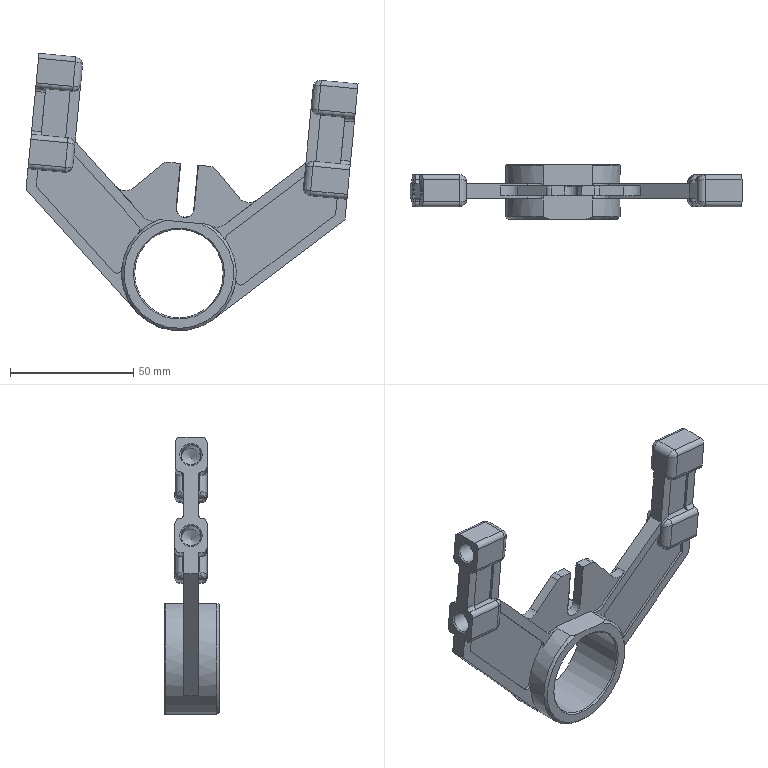Component | NX | DAZHOUZHICHENG | 1 solid | 192 faces | volume 42337 mm3 | plane 90 | cylinder 73 | spline 16 | cone 11 | torus 2 | commonest cylinder face diameters 4 x24 6 x24 3 x8 10 x6 0.4 x4 8 x4 46.5 x1 7 x1